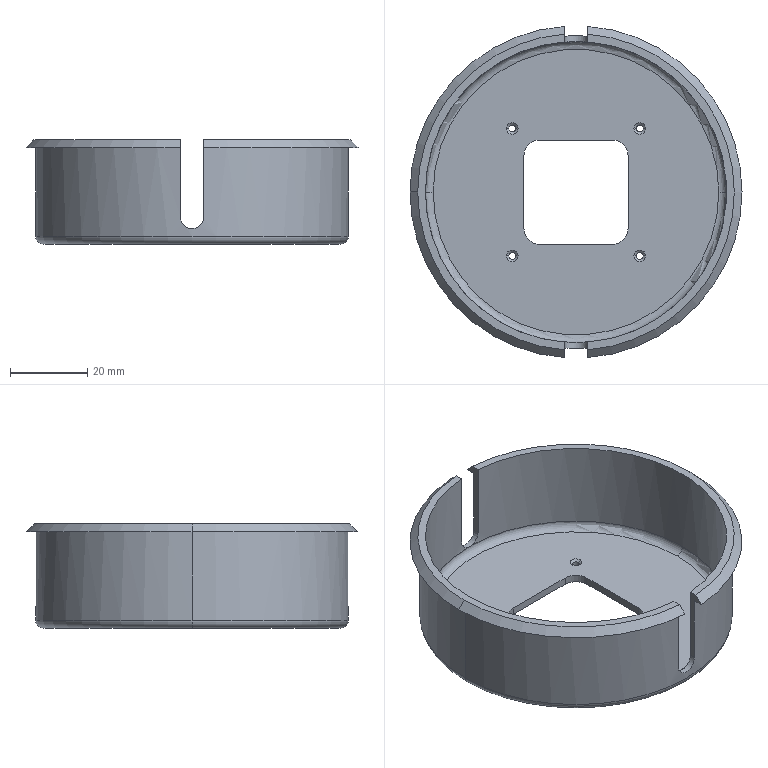Component | SolidWorks | GMotorCover-2 | 1 solid | 48 faces | volume 18550 mm3 | cylinder 19 | plane 14 | cone 11 | torus 4 | commonest cylinder face diameters 1.778 x8 8 x4 78 x3 81 x2 6 x2